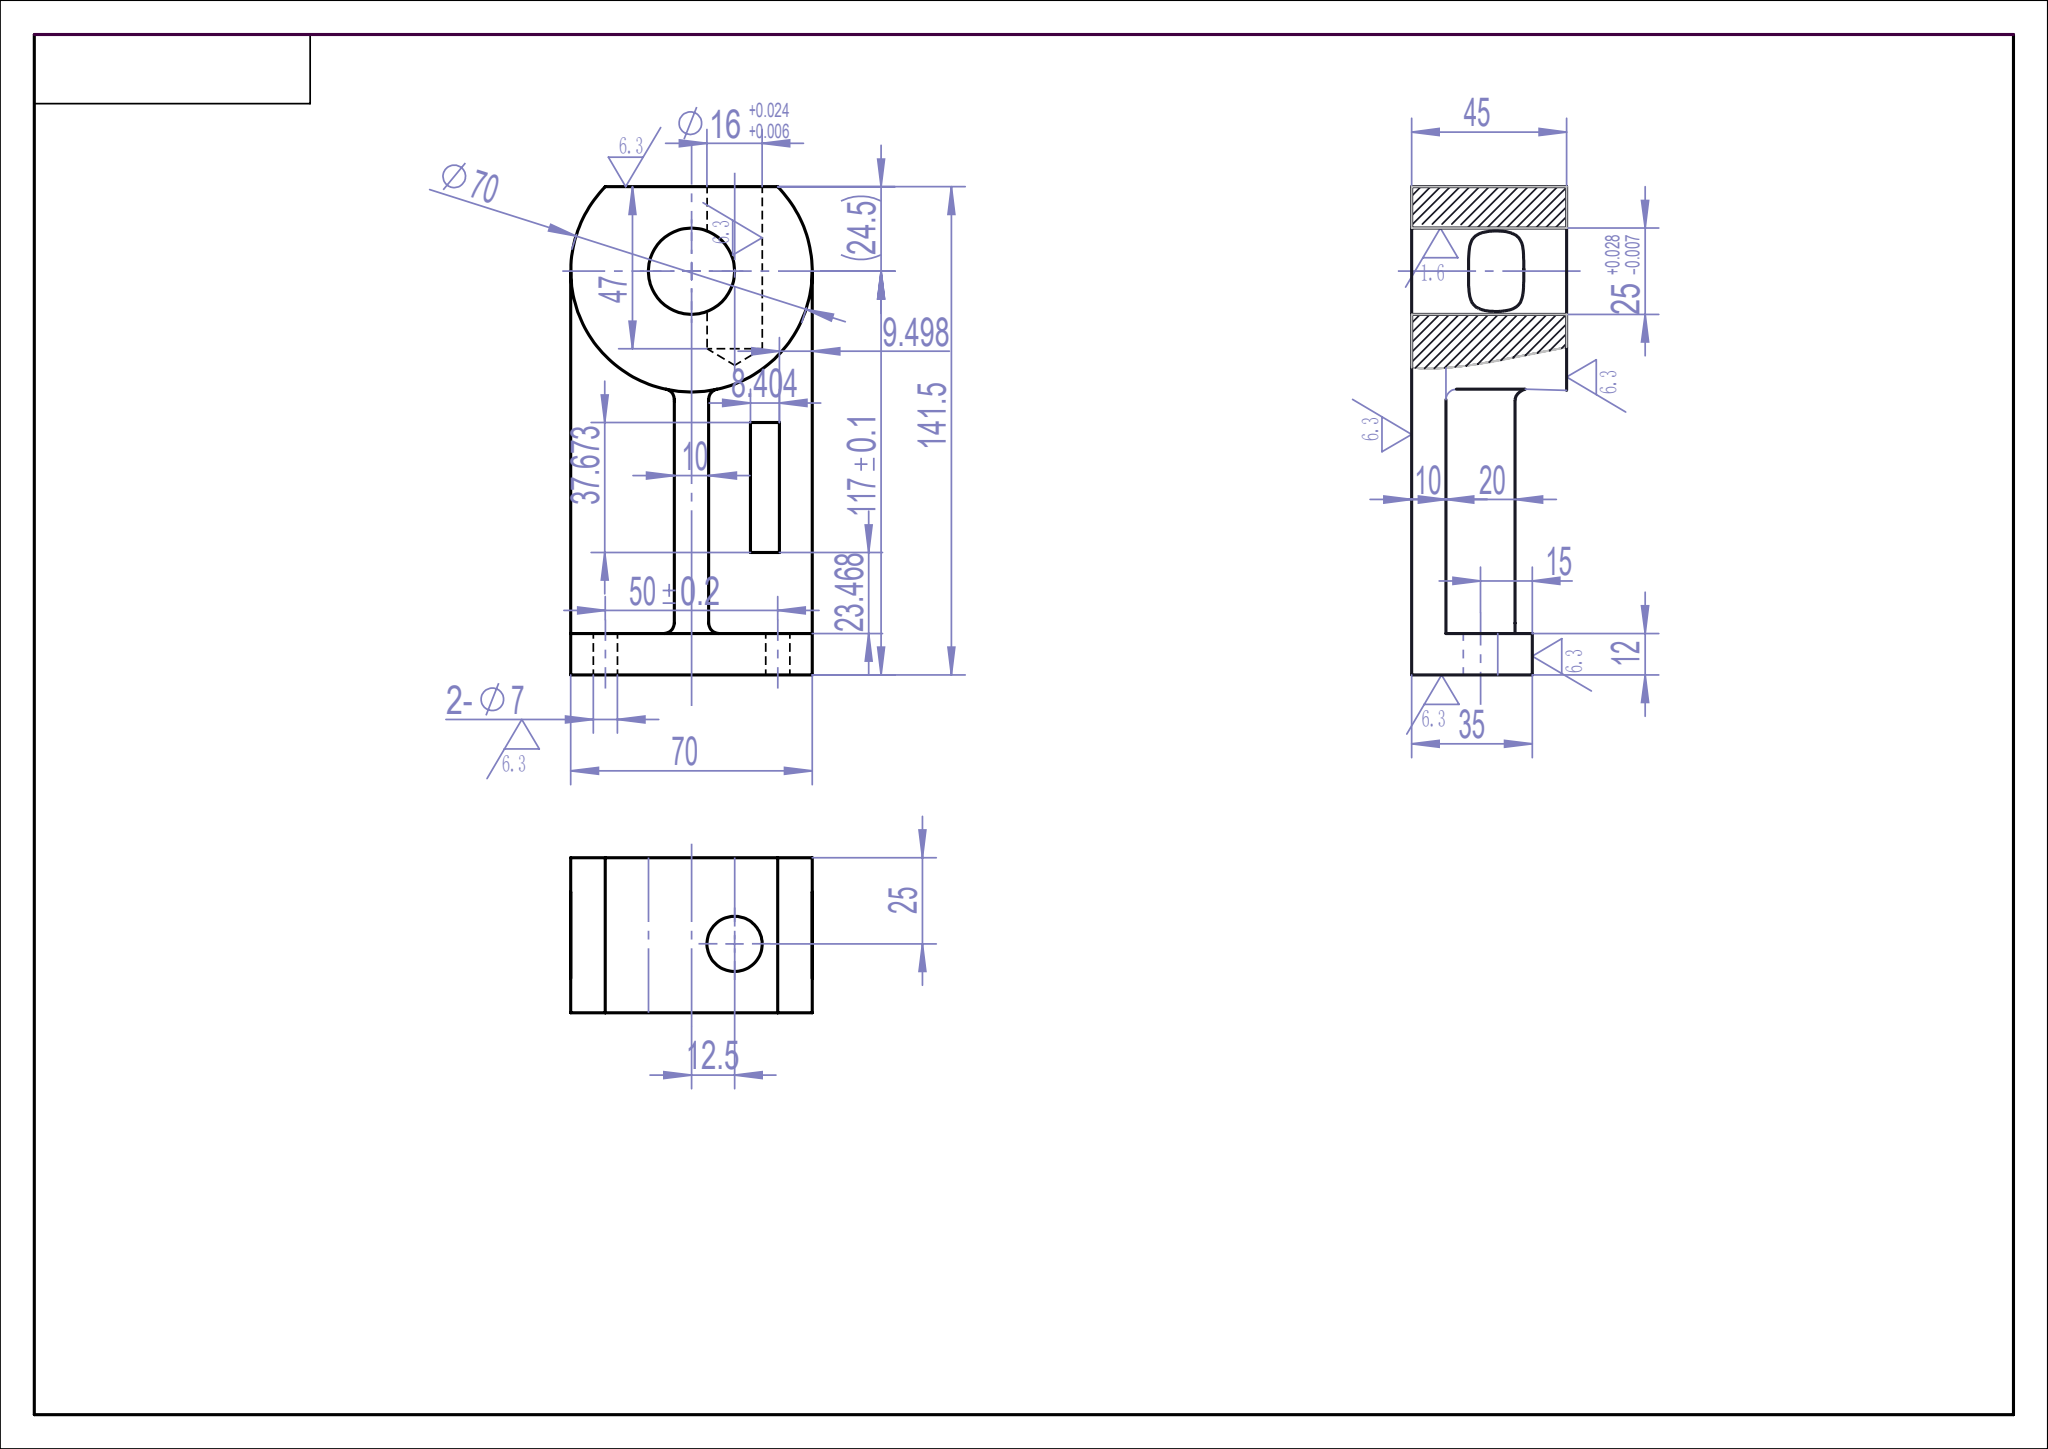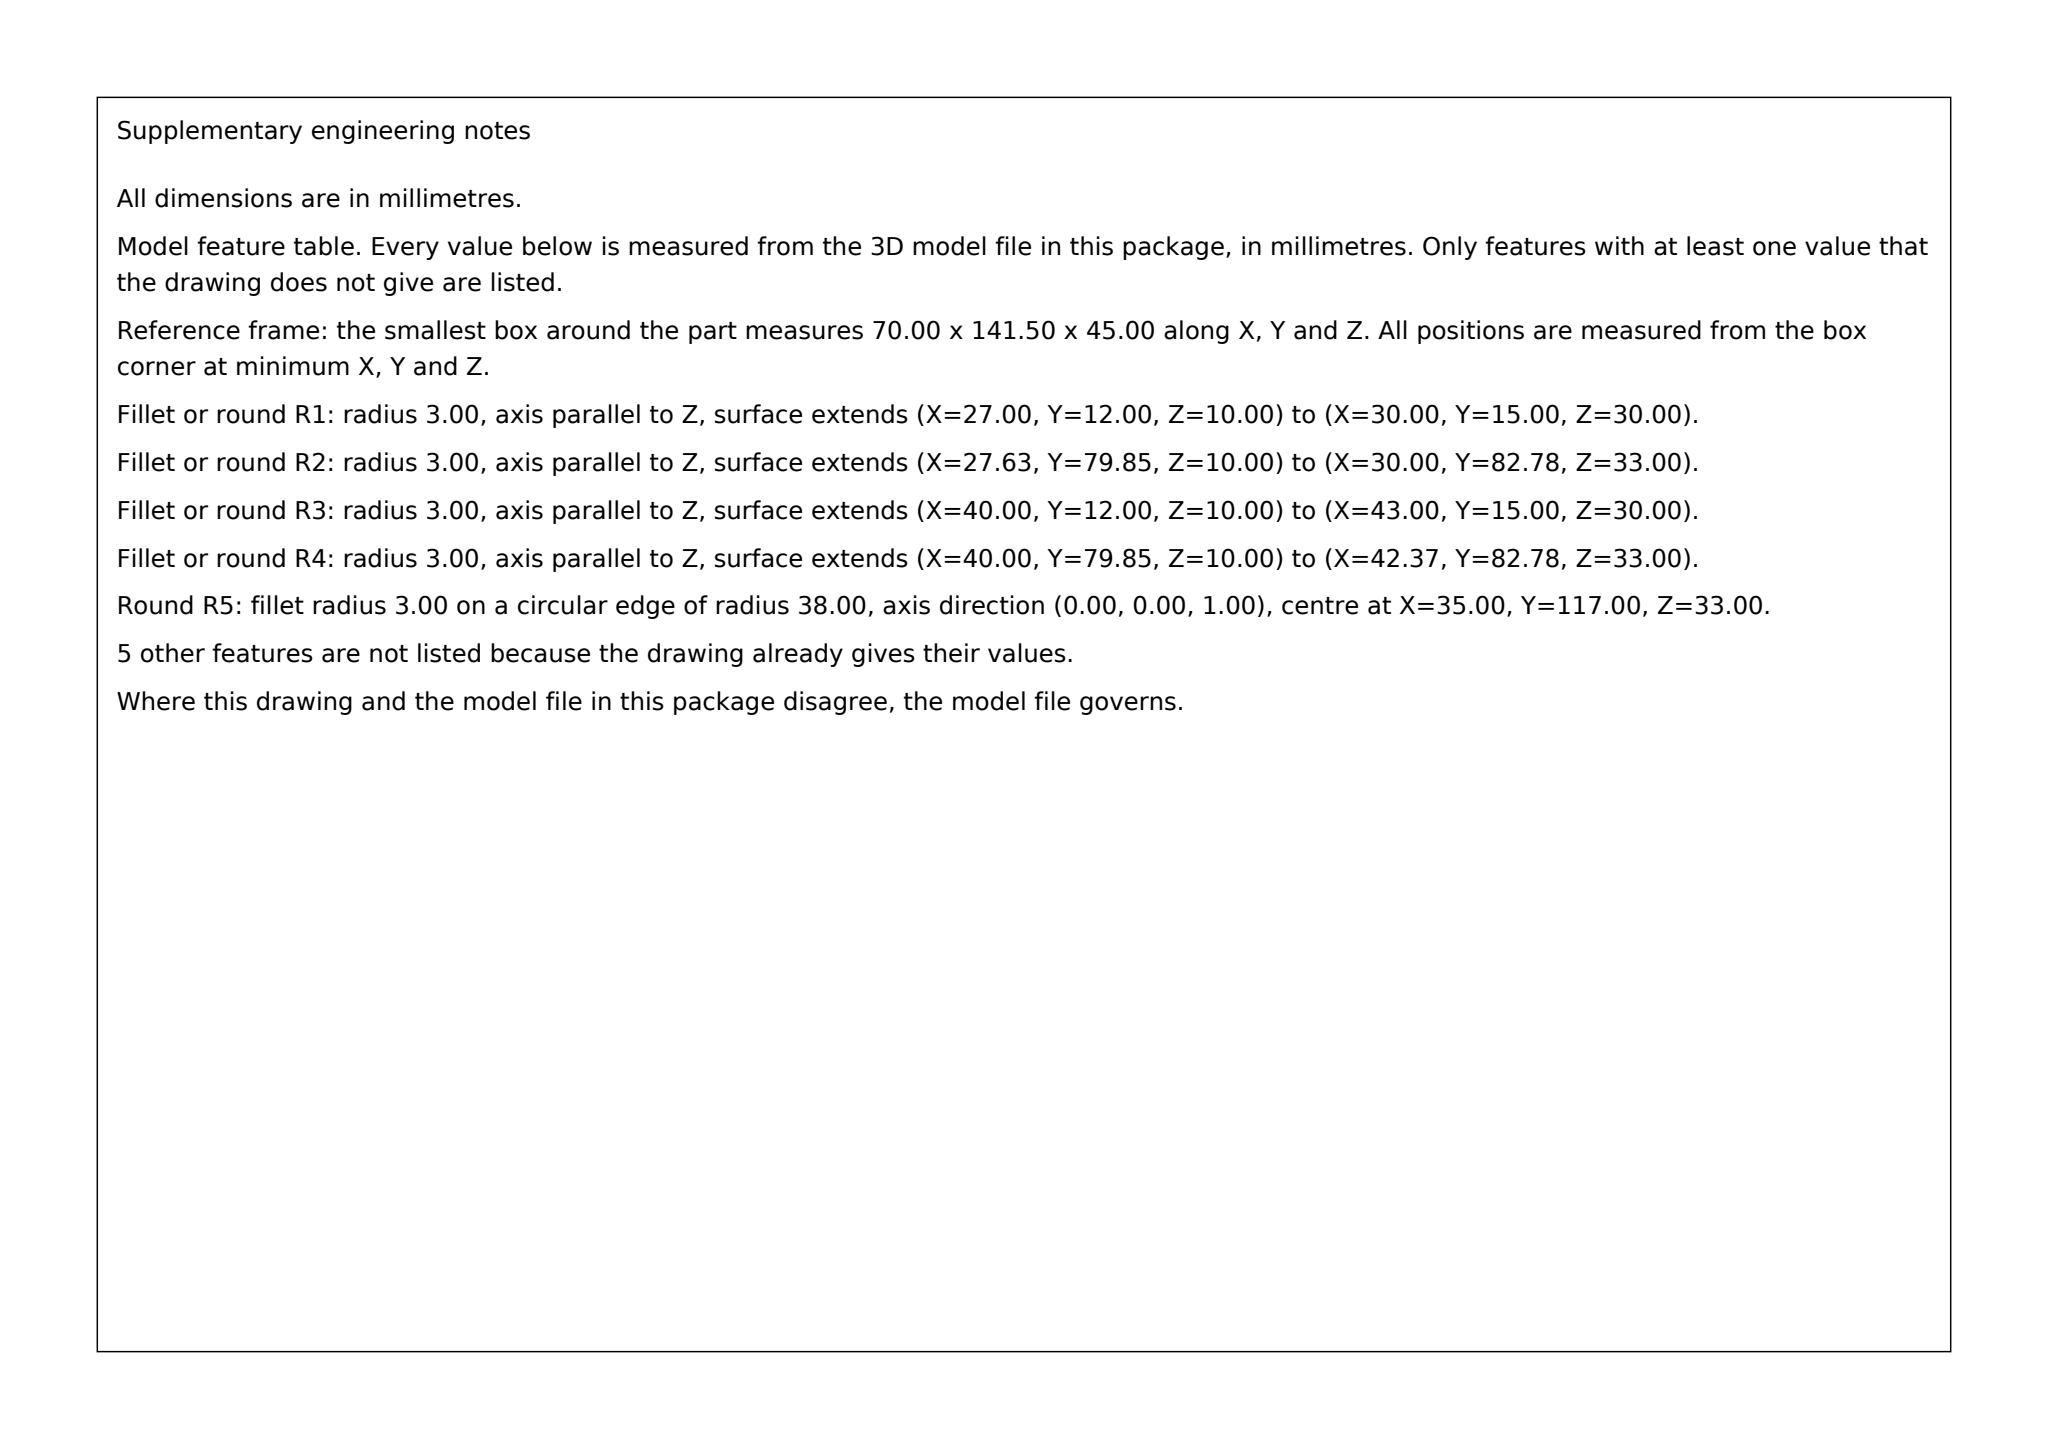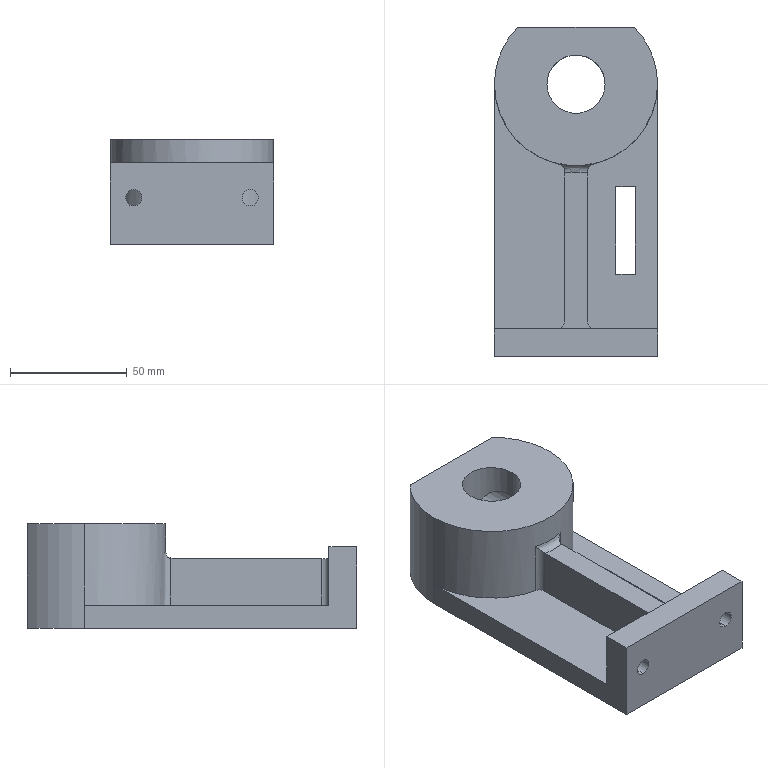Part | SolidWorks | mm | 1 solid | 36 faces | box 70 x 141.5 x 45 mm | volume 220353 mm3 | plane 17 | cylinder 16 | cone 2 | torus 1 | commonest cylinder face diameters 7 x4 6 x4 16 x3 70 x3 25 x2
build123d program:
from build123d import *

# Parameters (mm, degrees)
SKETCH1_R                      = 35
SKETCH1_R_2                    = 12.5
BOSS_EXTRUDE1_DEPTH            = 45
CUT_EXTRUDE1_START             = -45
CUT_EXTRUDE1_DEPTH             = 45
BOSS_EXTRUDE2_DEPTH            = 10
SKETCH5_W                      = 70
SKETCH5_H                      = 35
BOSS_EXTRUDE3_DEPTH            = 12
BOSS_EXTRUDE4_DEPTH            = 20
FILLET1_R                      = 3
F_16_0_16_DIAMETER_HOLE1_D     = 16
F_16_0_16_DIAMETER_HOLE1_DEPTH = 47
F_16_0_16_DIAMETER_HOLE1_TIP   = 4.807
SKETCH9_R                      = 3.5
CUT_EXTRUDE2_DEPTH             = 20
SKETCH10_W                     = 8.404
SKETCH10_H                     = 37.673
CUT_EXTRUDE3_DEPTH             = 59


with BuildPart() as part:
    # Sketch1 → Boss-Extrude1 (new body)
    with BuildSketch(Plane.XY):
        with Locations(Location((0, 0, 0), (0, 0, 180))):
            Circle(SKETCH1_R)
        with Locations(Location((0, 0, 0), (0, 0, 180))):
            Circle(SKETCH1_R_2, mode=Mode.SUBTRACT)
    extrude(amount=BOSS_EXTRUDE1_DEPTH)

    # Sketch3 → Cut-Extrude1 (cut)
    with BuildSketch(Plane.XY.offset(45).offset(CUT_EXTRUDE1_START)):
        with BuildLine():
            Line((-24.995, 24.5), (24.995, 24.5))
            ThreePointArc((24.995, 24.5), (0, 35), (-24.995, 24.5))
        make_face()
    extrude(amount=CUT_EXTRUDE1_DEPTH, mode=Mode.SUBTRACT)

    # Sketch4 → Boss-Extrude2 (add)
    with BuildSketch(Plane.XY):
        with BuildLine():
            Line((-35, 0), (-35, -117))
            Line((-35, -117), (35, -117))
            Line((35, -117), (35, 0))
            ThreePointArc((35, 0), (0, -35), (-35, 0))
        make_face()
    extrude(amount=BOSS_EXTRUDE2_DEPTH)

    # Sketch5 → Boss-Extrude3 (add)
    with BuildSketch(Plane.XZ.offset(117)):
        with Locations((0, 17.5)):
            Rectangle(SKETCH5_W, SKETCH5_H)
    extrude(amount=-BOSS_EXTRUDE3_DEPTH)

    # Sketch6 → Boss-Extrude4 (add)
    with BuildSketch(Plane.XY.offset(10)):
        with BuildLine():
            Line((-5, -34.641), (-5, -105))
            Line((-5, -105), (5, -105))
            Line((5, -105), (5, -34.641))
            ThreePointArc((5, -34.641), (0, -35), (-5, -34.641))
        make_face()
    extrude(amount=BOSS_EXTRUDE4_DEPTH)

    # Fillet1
    fillet1_edges = [part.edges().sort_by_distance(p)[0] for p in [
        (5, -34.641, 20),
        (-5, -34.641, 20),
        (-5, -105, 20),
        (5, -105, 20),
        (0, -35, 30),
    ]]
    fillet(fillet1_edges, radius=FILLET1_R)

    # 16.0 _16_ Diameter Hole1
    with Locations(Plane(origin=(12.5, 24.5, 25), x_dir=(0, 0, 1), z_dir=(0, 1, 0))):
        with Locations((0, 0)):
            Hole(F_16_0_16_DIAMETER_HOLE1_D / 2, depth=F_16_0_16_DIAMETER_HOLE1_DEPTH)
            with Locations((0, 0, -(F_16_0_16_DIAMETER_HOLE1_DEPTH + F_16_0_16_DIAMETER_HOLE1_TIP / 2))):  # 118° drill point
                Cone(0, F_16_0_16_DIAMETER_HOLE1_D / 2, F_16_0_16_DIAMETER_HOLE1_TIP, mode=Mode.SUBTRACT)

    # Sketch9 → Cut-Extrude2 (cut)
    with BuildSketch(Plane(origin=(0, -105, 0), x_dir=(1, 0, 0), z_dir=(0, 1, 0))):
        with Locations(Location((-25, -20, 0), (0, 0, 270))):
            Circle(SKETCH9_R)
        with Locations(Location((25, -20, 0), (0, 0, 270))):
            Circle(SKETCH9_R)
    extrude(amount=-CUT_EXTRUDE2_DEPTH, mode=Mode.SUBTRACT)

    # Sketch10 → Cut-Extrude3 (cut)
    with BuildSketch(Plane.XY.offset(10)):
        with Locations((21.3, -62.696)):
            Rectangle(SKETCH10_W, SKETCH10_H)
    extrude(amount=-CUT_EXTRUDE3_DEPTH, mode=Mode.SUBTRACT)


solid = part.part